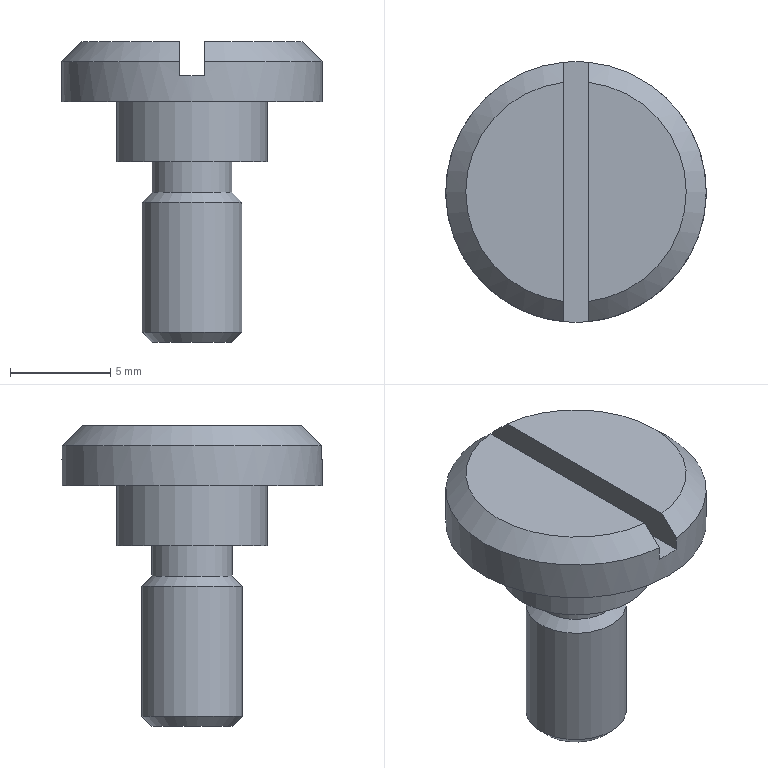Component | NX | DRILL_BUSHING_SCREW_2 | 1 solid | 16 faces | volume 649 mm3 | plane 8 | cylinder 4 | cone 4 | commonest cylinder face diameters 5 x1 4 x1 7.5 x1 13 x1